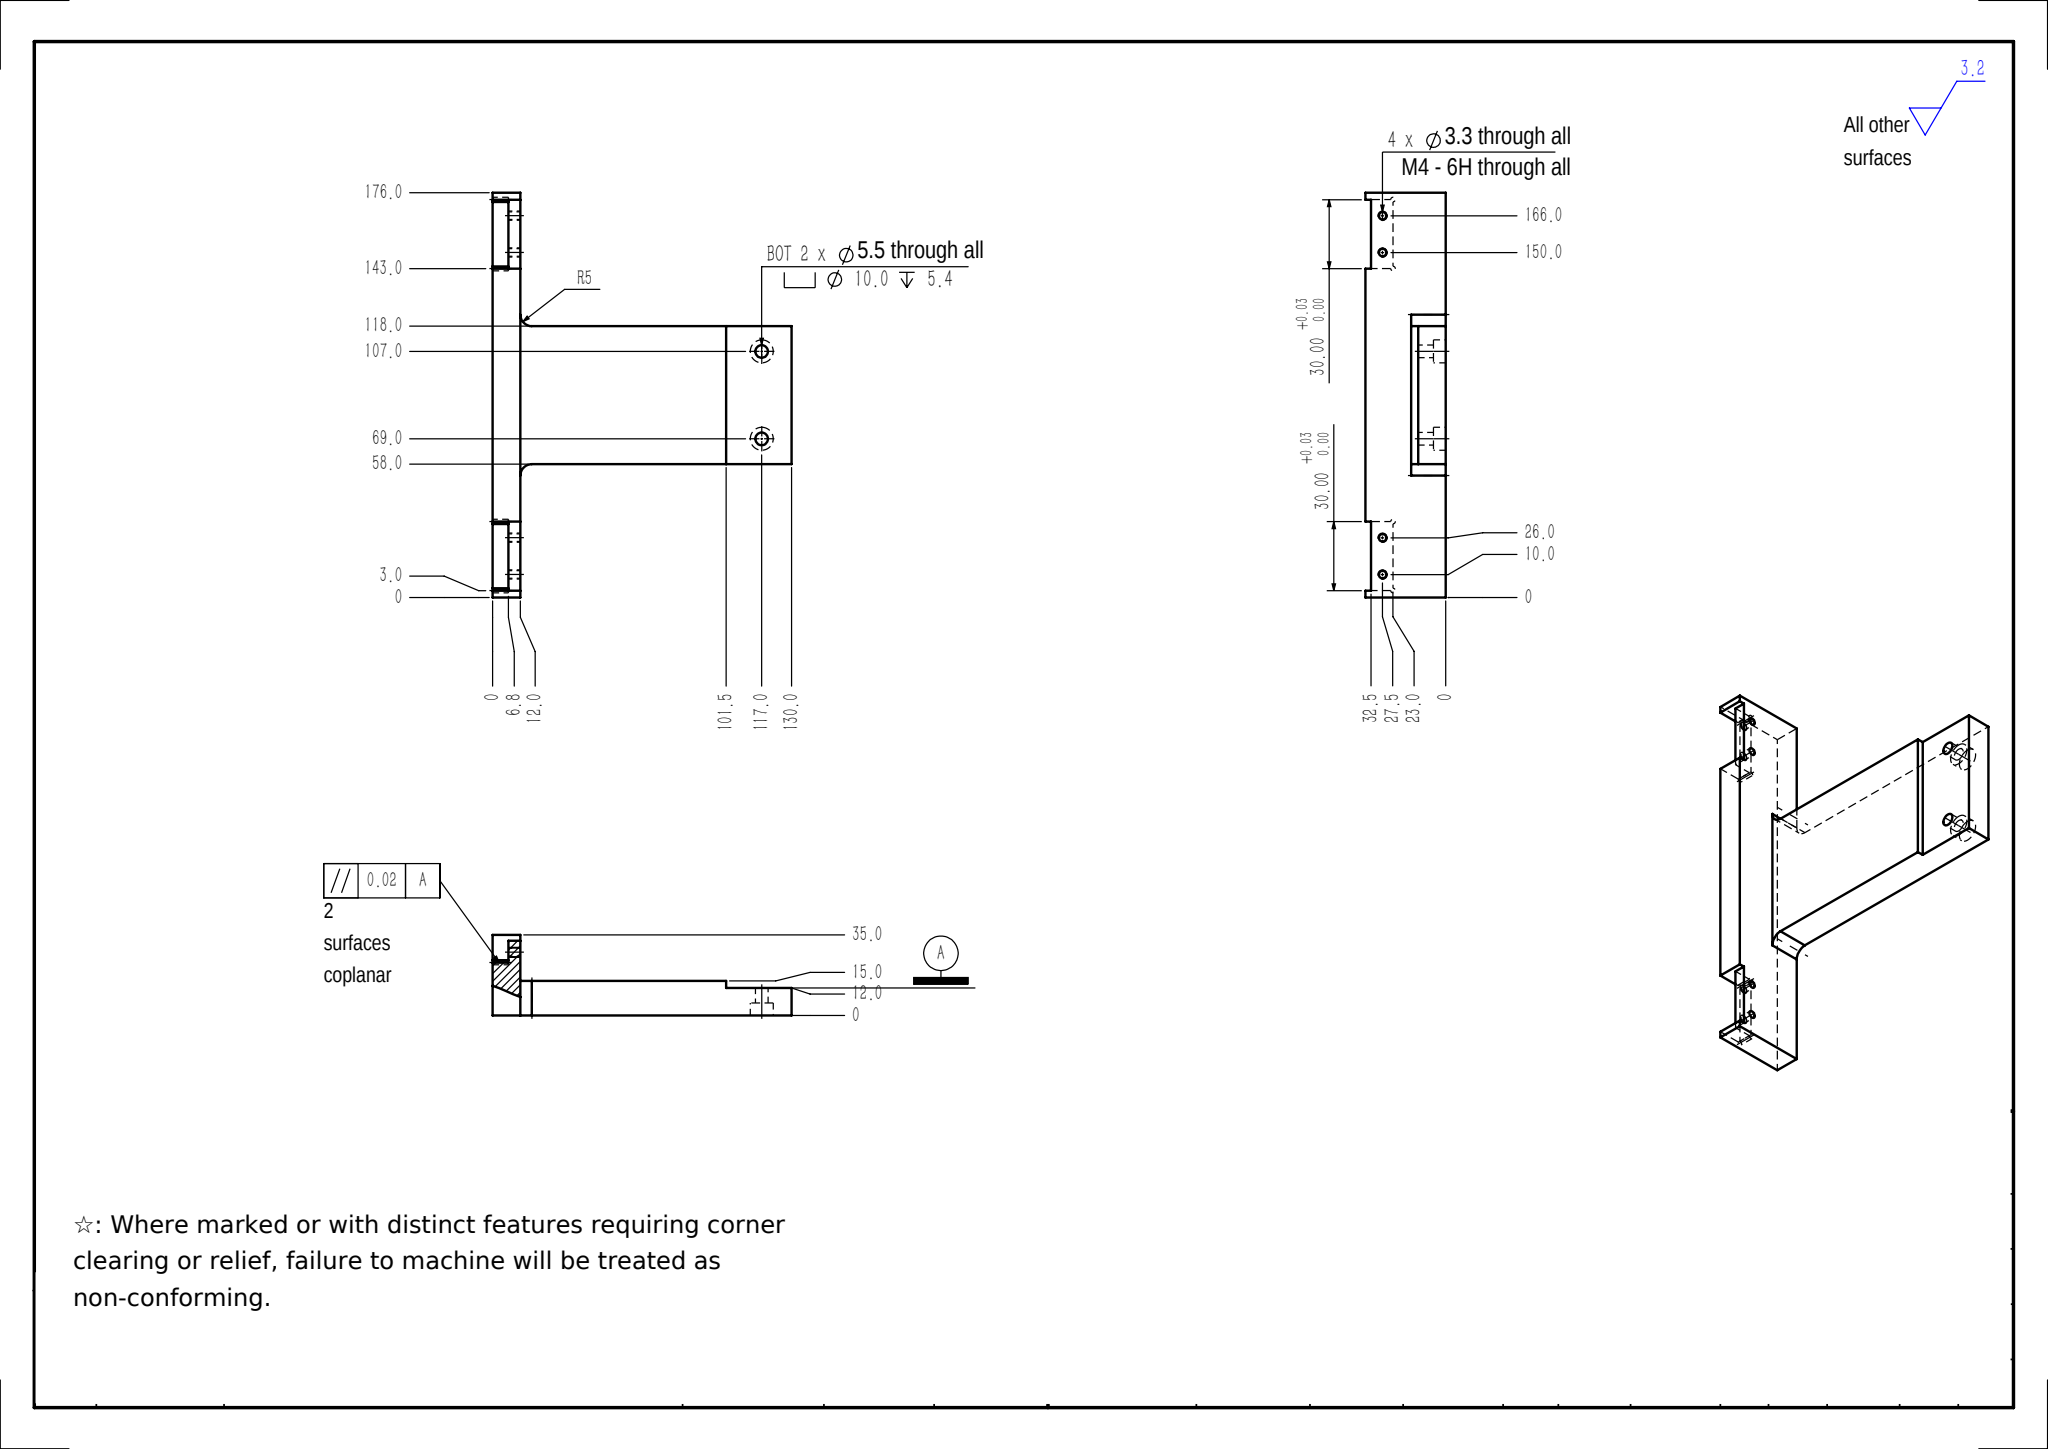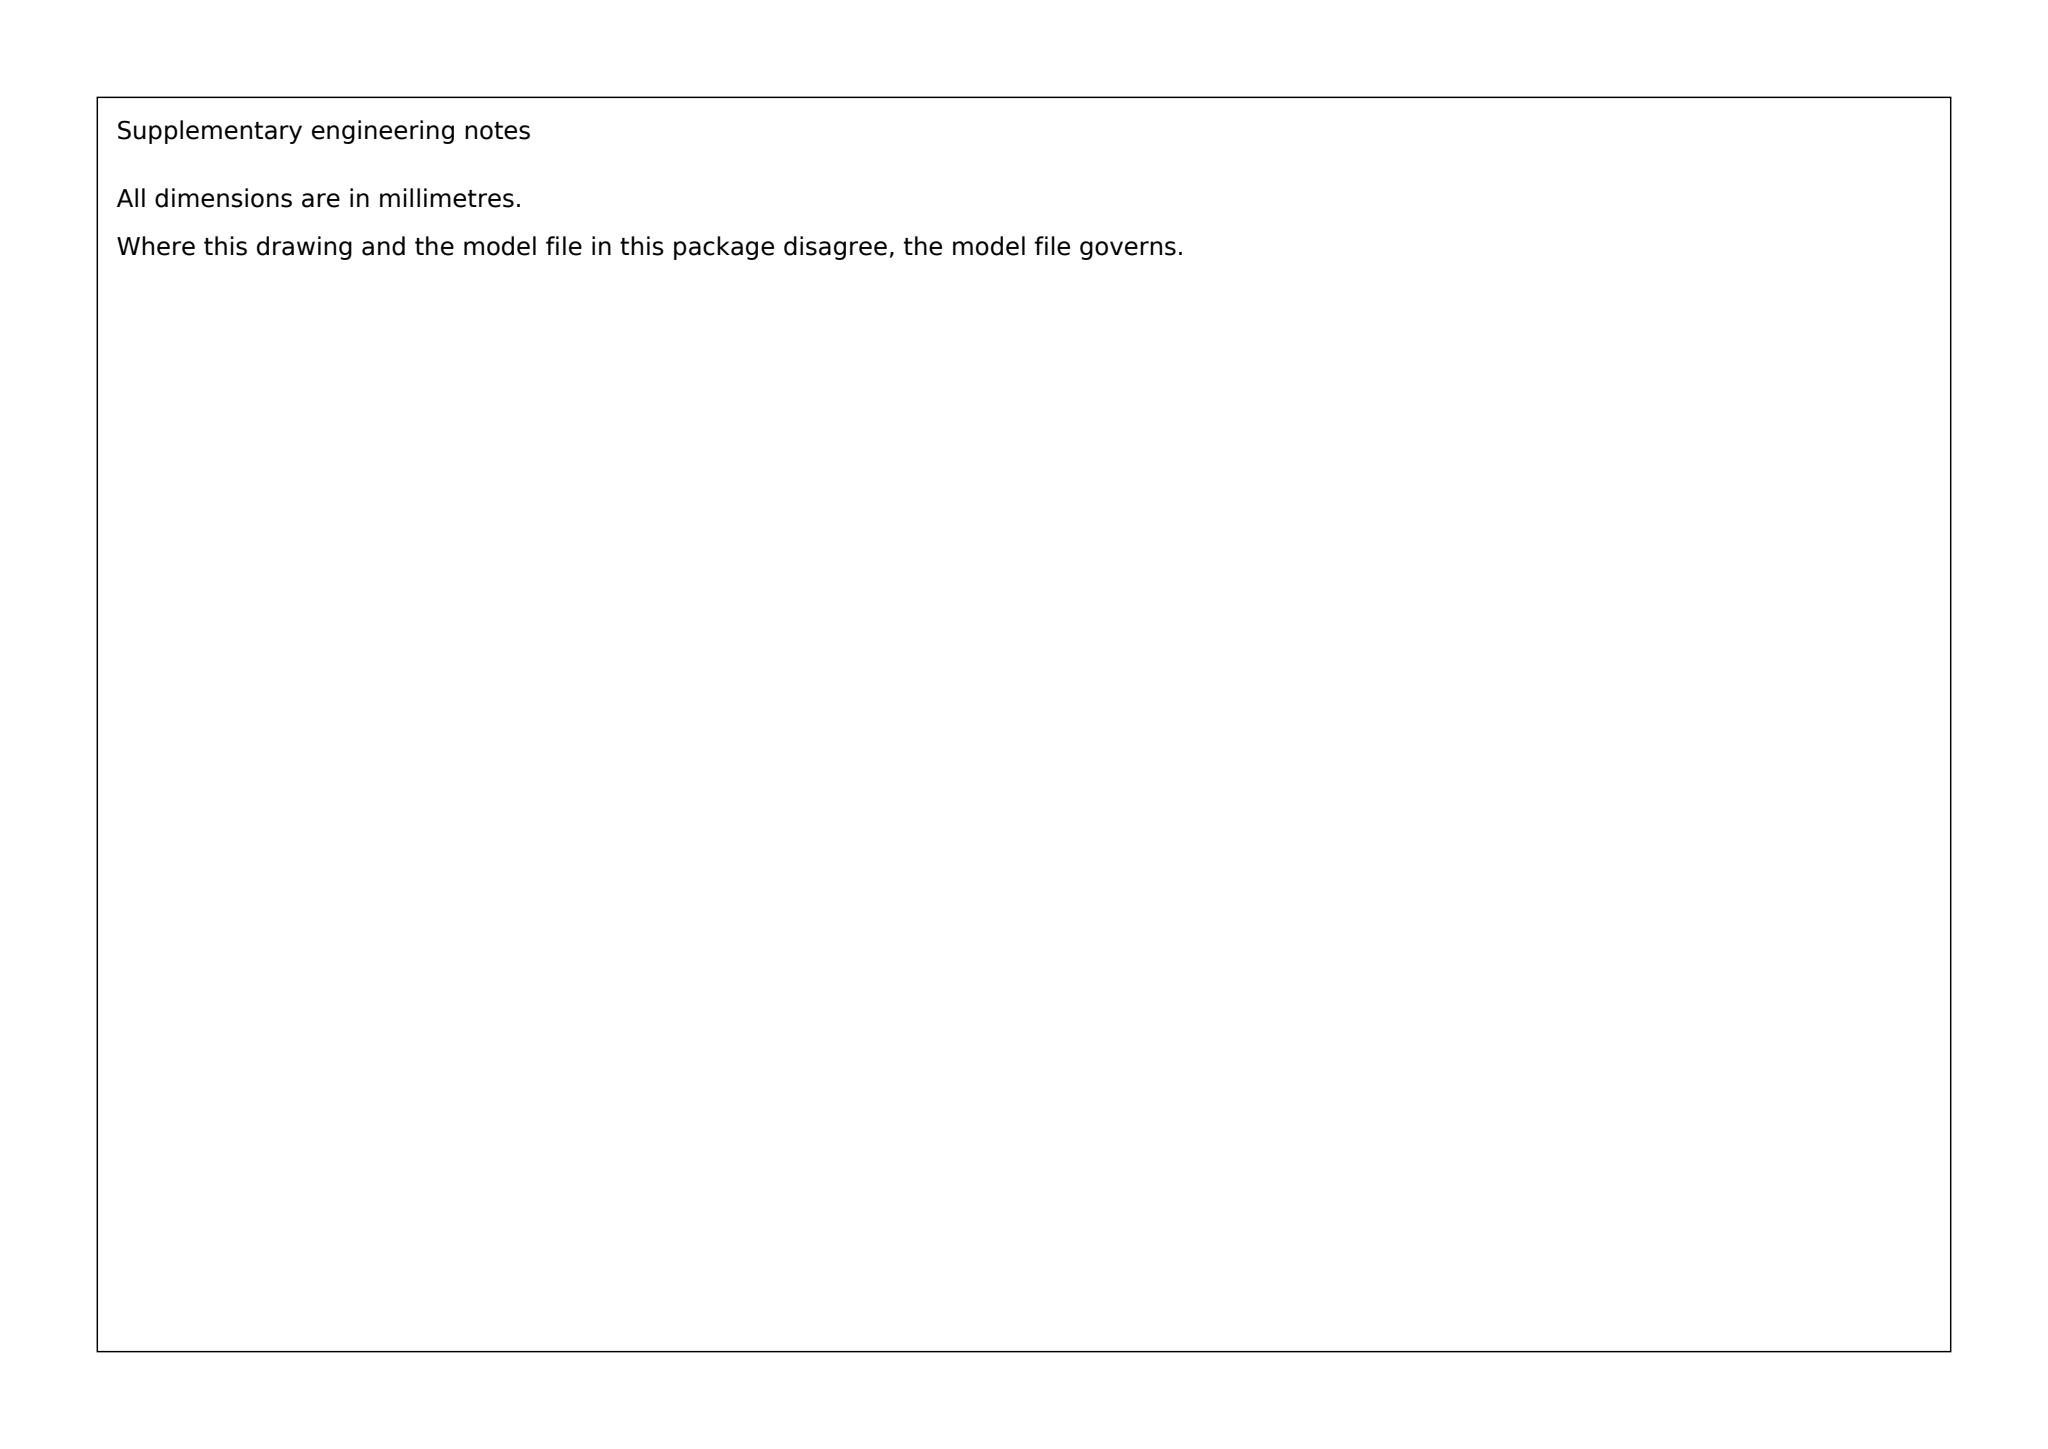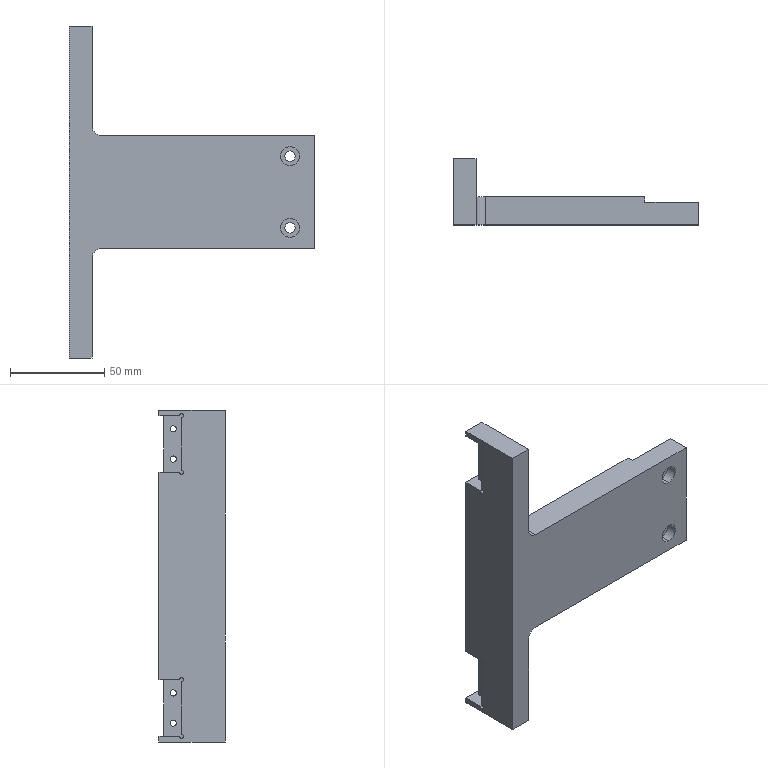Part | SolidWorks | mm | 1 solid | 52 faces | box 130 x 35 x 176 mm | volume 168071 mm3 | cylinder 26 | plane 26 | commonest cylinder face diameters 3.3 x8 2 x8 10 x6 5.5 x4
build123d program:
from build123d import *

# Parameters (mm, degrees)
SKETCH1_W                                       = 12
SKETCH1_H                                       = 35
BOSS_EXTRUDE1_DEPTH                             = 88
SKETCH13_W                                      = 176
SKETCH13_H                                      = 15
BOSS_EXTRUDE2_DEPTH                             = 118
SKETCH7_W                                       = 30
SKETCH7_H                                       = 12
CUT_EXTRUDE3_DEPTH                              = 6.8
SKETCH8_R                                       = 1
CUT_EXTRUDE4_DEPTH                              = 6.8
SKETCH15_W                                      = 28.5
SKETCH15_H                                      = 236
CUT_EXTRUDE6_DEPTH                              = 3
M5_HEX_SOCKET_HEAD_CAP_SCREW_CBORE1_D           = 5.5
M5_HEX_SOCKET_HEAD_CAP_SCREW_CBORE1_CBORE_D     = 10
M5_HEX_SOCKET_HEAD_CAP_SCREW_CBORE1_CBORE_DEPTH = 5.4
SKETCH19_W                                      = 30
SKETCH19_H                                      = 2.5
CUT_EXTRUDE8_DEPTH                              = 153.409
M4_TAPPED_HOLE1_D                               = 3.3
CUT_EXTRUDE9_DEPTH                              = 154.362


with BuildPart() as part:
    # Sketch1 → Boss-Extrude1 (new, symmetric)
    with BuildSketch(Plane.XY):
        Rectangle(SKETCH1_W, SKETCH1_H)
    extrude(amount=BOSS_EXTRUDE1_DEPTH, both=True)

    # Sketch13 → Boss-Extrude2 (add)
    with BuildSketch(Plane(origin=(6, 0, 0), x_dir=(0, 0, -1), z_dir=(1, 0, 0))):
        with Locations((0, -10)):
            Rectangle(SKETCH13_W, SKETCH13_H)
    extrude(amount=BOSS_EXTRUDE2_DEPTH)

    # Sketch7 → Cut-Extrude3 (cut)
    with BuildSketch(Plane.ZY.offset(6)):
        with Locations((70, 11.5)):
            Rectangle(SKETCH7_W, SKETCH7_H)
        with Locations((-70, 11.5)):
            Rectangle(SKETCH7_W, SKETCH7_H)
    extrude(amount=-CUT_EXTRUDE3_DEPTH, mode=Mode.SUBTRACT)

    # Sketch8 → Cut-Extrude4 (cut)
    with BuildSketch(Plane.ZY.offset(6)):
        with Locations((85, 5.5)):
            Circle(SKETCH8_R)
        with Locations((55, 5.5)):
            Circle(SKETCH8_R)
    cut_extrude4 = extrude(amount=-CUT_EXTRUDE4_DEPTH, mode=Mode.SUBTRACT)

    # Sketch15 → Cut-Extrude6 (cut)
    with BuildSketch(Plane(origin=(0, -2.5, 0), x_dir=(1, 0, 0), z_dir=(0, 1, 0))):
        with Locations((109.75, 0)):
            Rectangle(SKETCH15_W, SKETCH15_H)
    extrude(amount=-CUT_EXTRUDE6_DEPTH, mode=Mode.SUBTRACT)

    # M5 Hex Socket Head Cap Screw CBORE1 (through all)
    with Locations(Plane(origin=(0, -17.5, 0), x_dir=(-1, 0, 0), z_dir=(0, -1, 0))):
        with Locations((-111, 19), (-111, -19)):
            CounterBoreHole(M5_HEX_SOCKET_HEAD_CAP_SCREW_CBORE1_D / 2, M5_HEX_SOCKET_HEAD_CAP_SCREW_CBORE1_CBORE_D / 2, M5_HEX_SOCKET_HEAD_CAP_SCREW_CBORE1_CBORE_DEPTH)

    # Sketch19 → Cut-Extrude8 (cut, through all)
    with BuildSketch(Plane.ZY.offset(-0.8)):
        with Locations((70, 16.25)):
            Rectangle(SKETCH19_W, SKETCH19_H)
    cut_extrude8 = extrude(amount=-CUT_EXTRUDE8_DEPTH, mode=Mode.SUBTRACT)

    # M4 Tapped Hole1 (through all)
    with Locations(Plane.ZY.offset(-0.8)):
        with Locations((78, 10), (62, 10)):
            m4_tapped_hole1 = Hole(M4_TAPPED_HOLE1_D / 2)

    # Mirror1: Cut-Extrude4, Cut-Extrude8, M4 Tapped Hole1 across plane
    add(cut_extrude4.mirror(Plane.XY), mode=Mode.SUBTRACT)
    add(cut_extrude8.mirror(Plane.XY), mode=Mode.SUBTRACT)
    add(m4_tapped_hole1.mirror(Plane.XY), mode=Mode.SUBTRACT)

    # Sketch22 → Cut-Extrude9 (cut, through all)
    with BuildSketch(Plane(origin=(0, -2.5, 0), x_dir=(1, 0, 0), z_dir=(0, 1, 0))):
        with BuildLine():
            Line((124, 88), (6, 88))
            Line((6, 88), (6, 35))
            ThreePointArc((6, 35), (7.464, 31.464), (11, 30))
            Line((11, 30), (124, 30))
            Line((124, 30), (124, 88))
        make_face()
        with BuildLine():
            Line((6, -88), (6, -35))
            ThreePointArc((6, -35), (7.464, -31.464), (11, -30))
            Line((11, -30), (124, -30))
            Line((124, -30), (124, -88))
            Line((124, -88), (6, -88))
        make_face()
    extrude(amount=-CUT_EXTRUDE9_DEPTH, mode=Mode.SUBTRACT)


solid = part.part